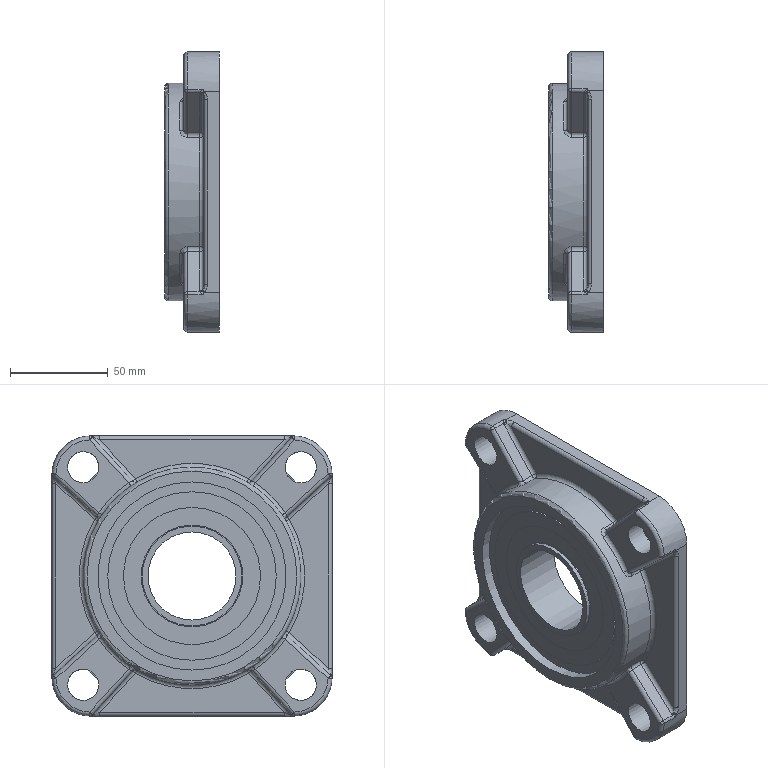Component | NX | BEARING_HOUSING_1 | 1 solid | 222 faces | volume 264029 mm3 | cylinder 72 | plane 61 | spline 48 | torus 25 | sphere 16 | commonest cylinder face diameters 4 x40 20 x8 16 x4 40 x4 143 x4 51 x2 111 x1 52 x1